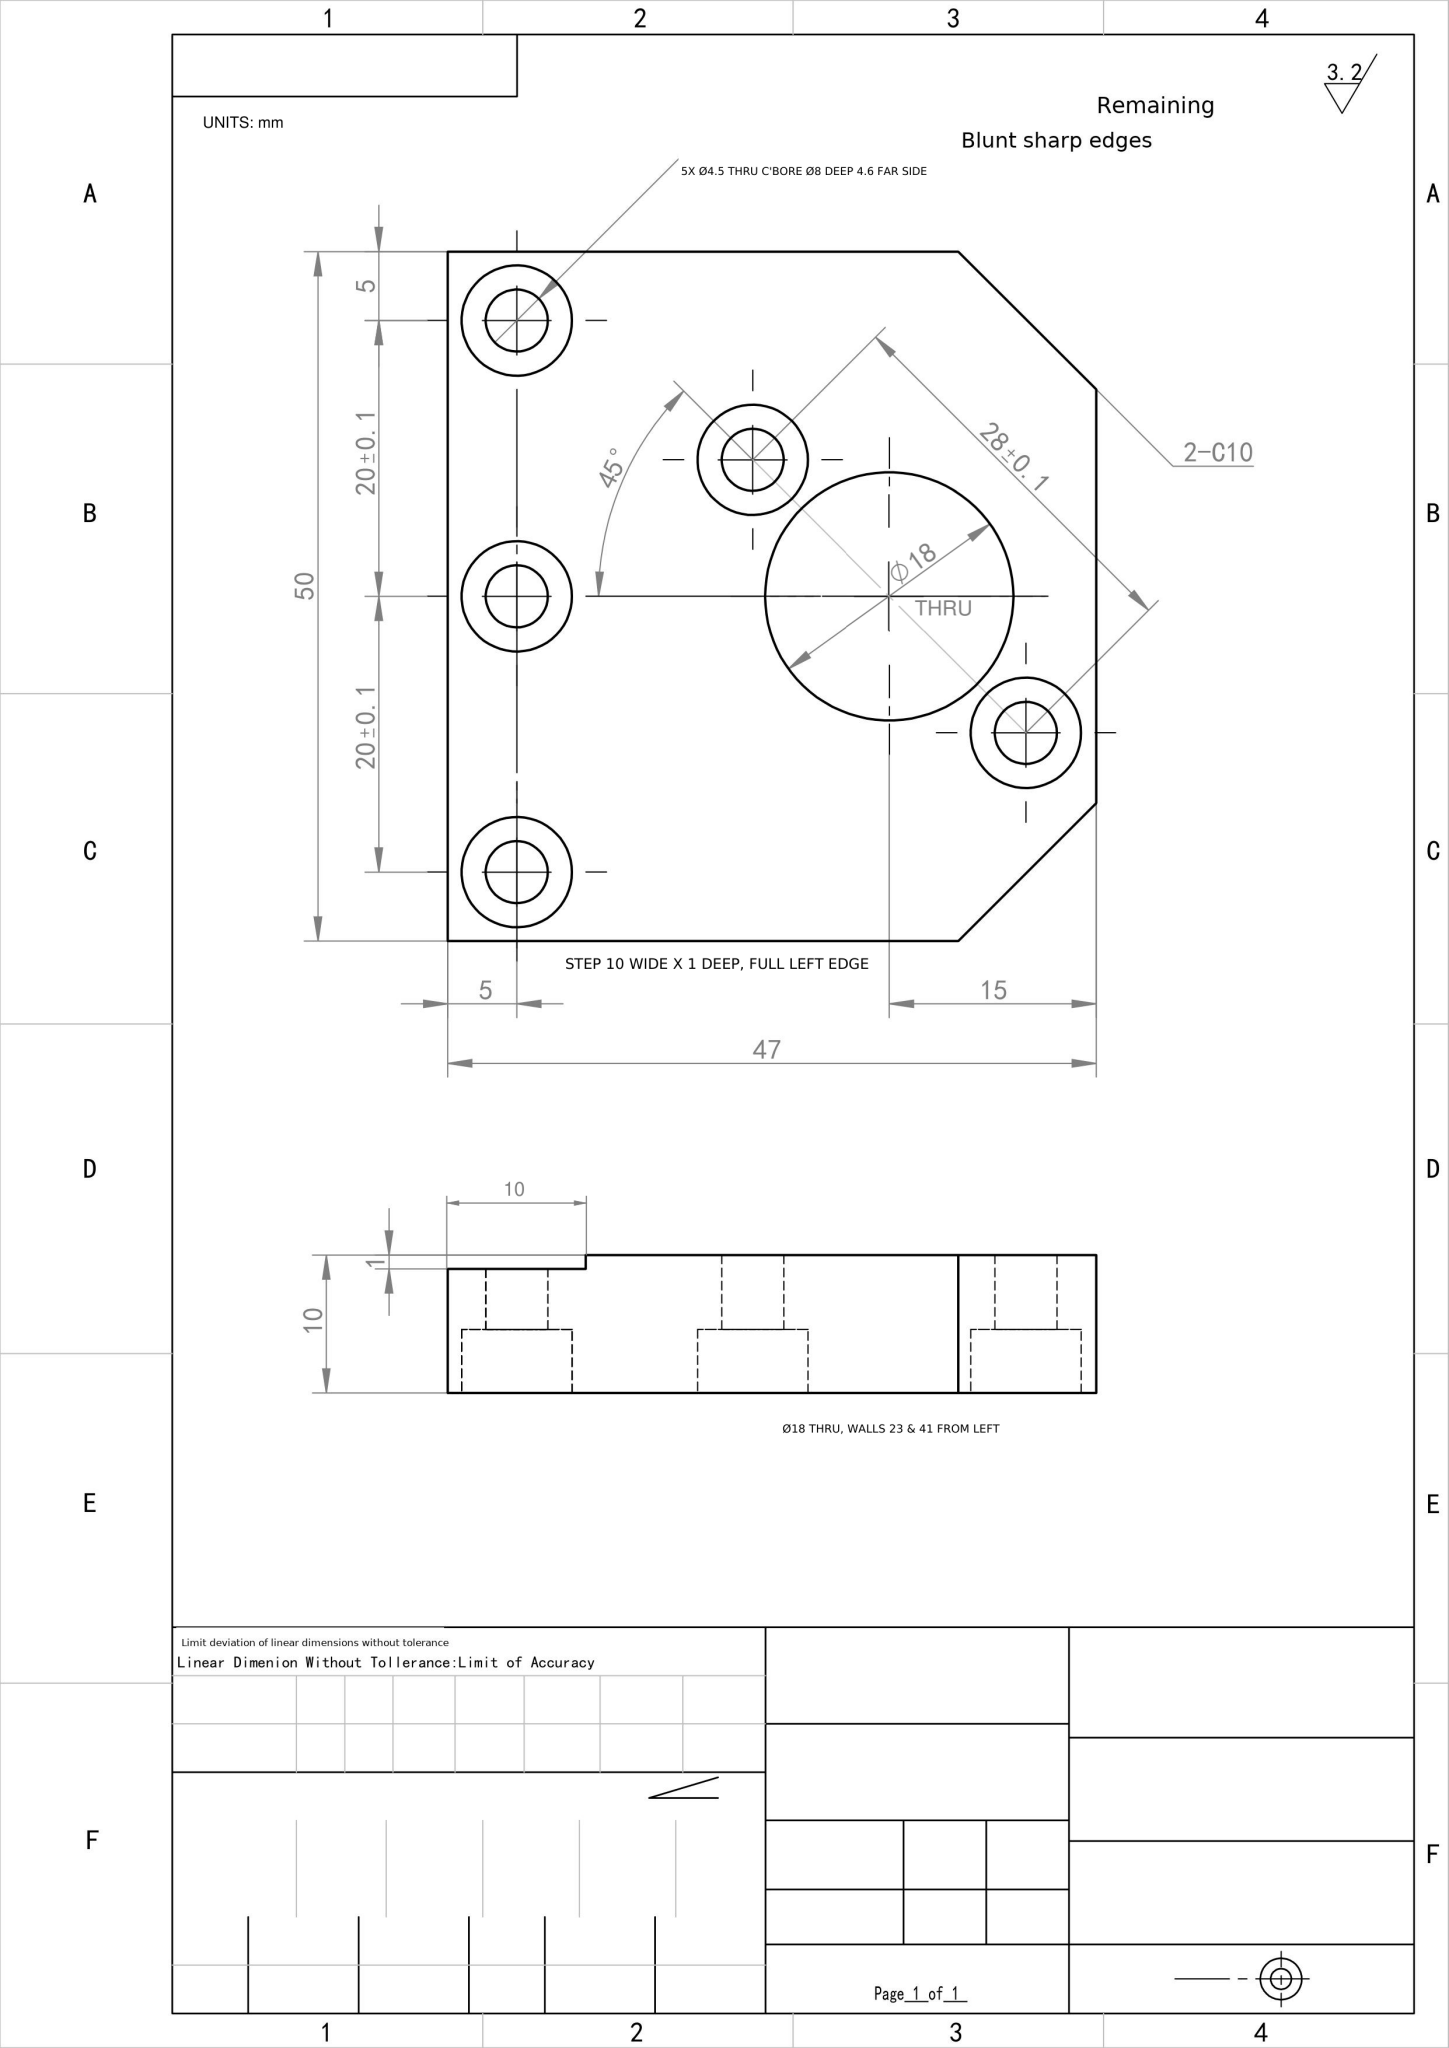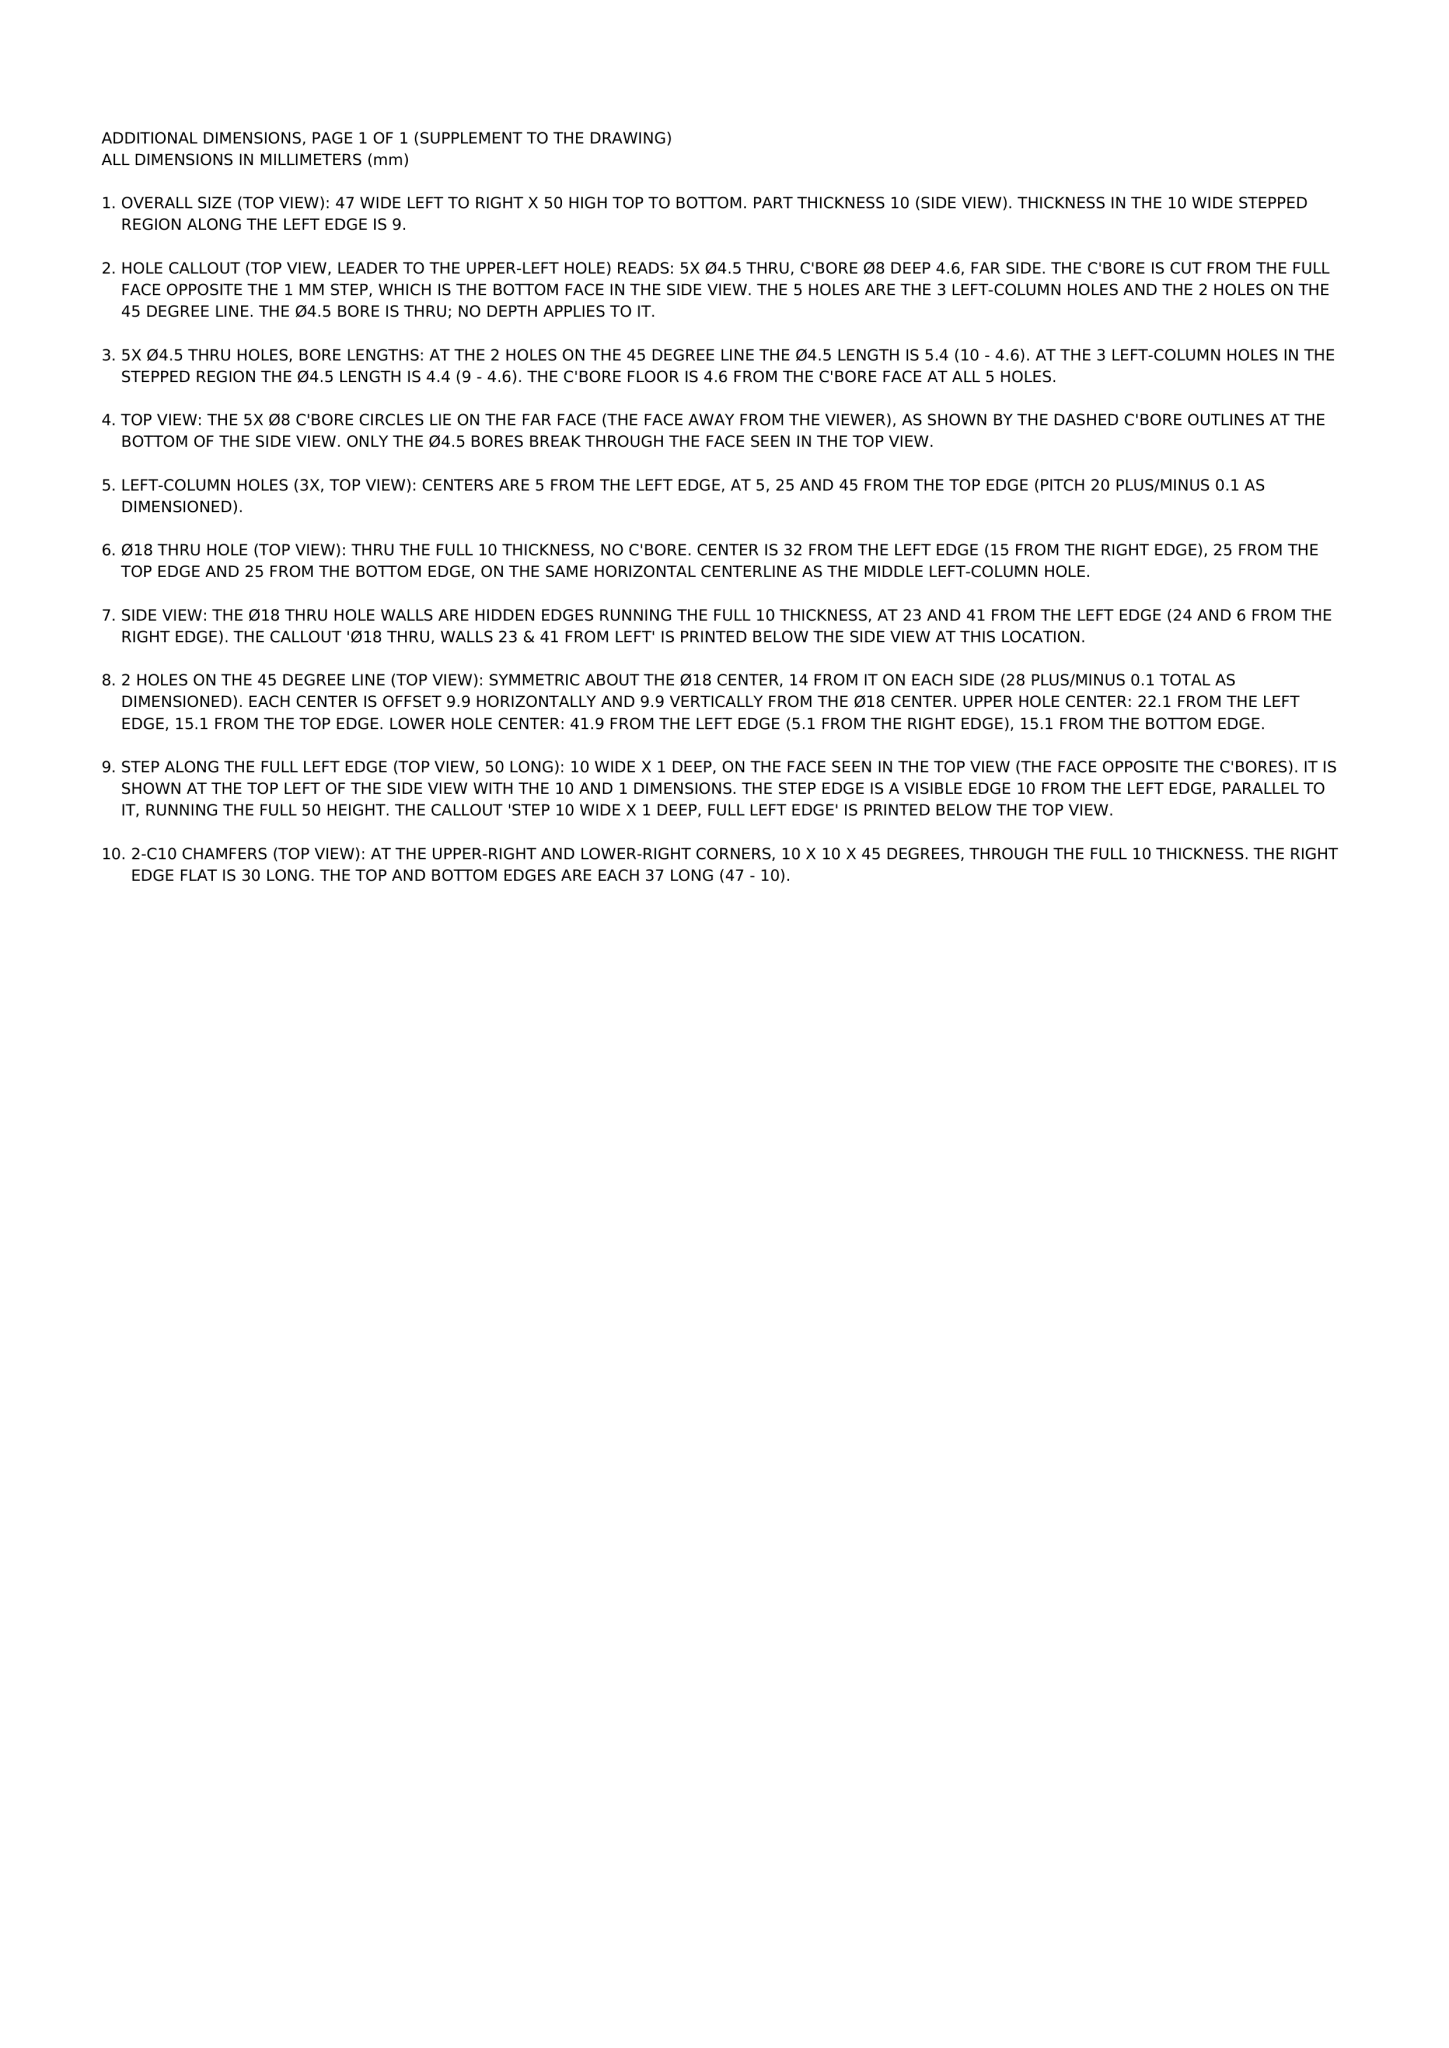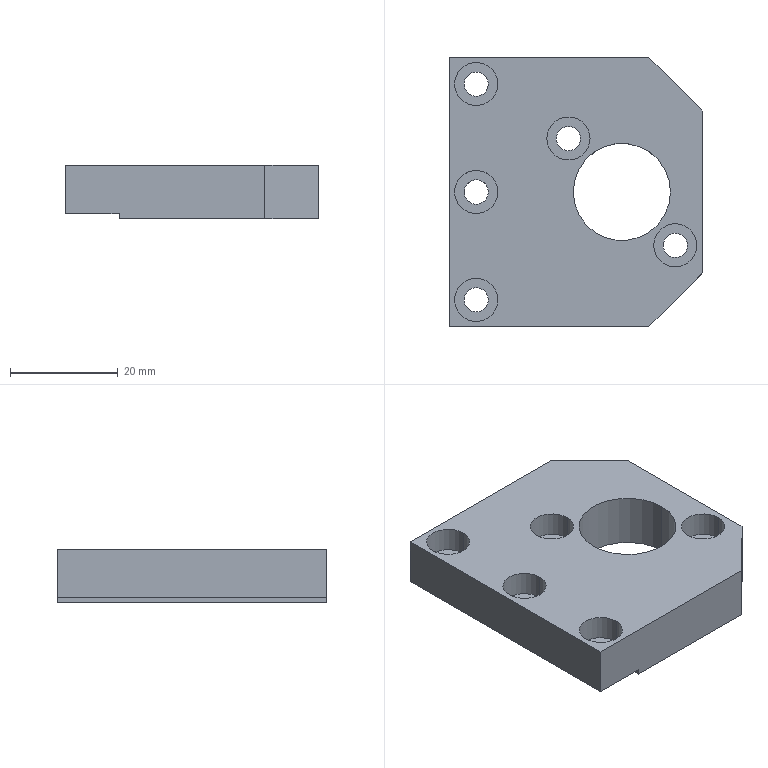Part | NX | mm | 1 solid | 37 faces | box 47 x 50 x 10 mm | volume 17918 mm3 | cylinder 22 | plane 15 | commonest cylinder face diameters 8 x10 4.5 x10 18 x2